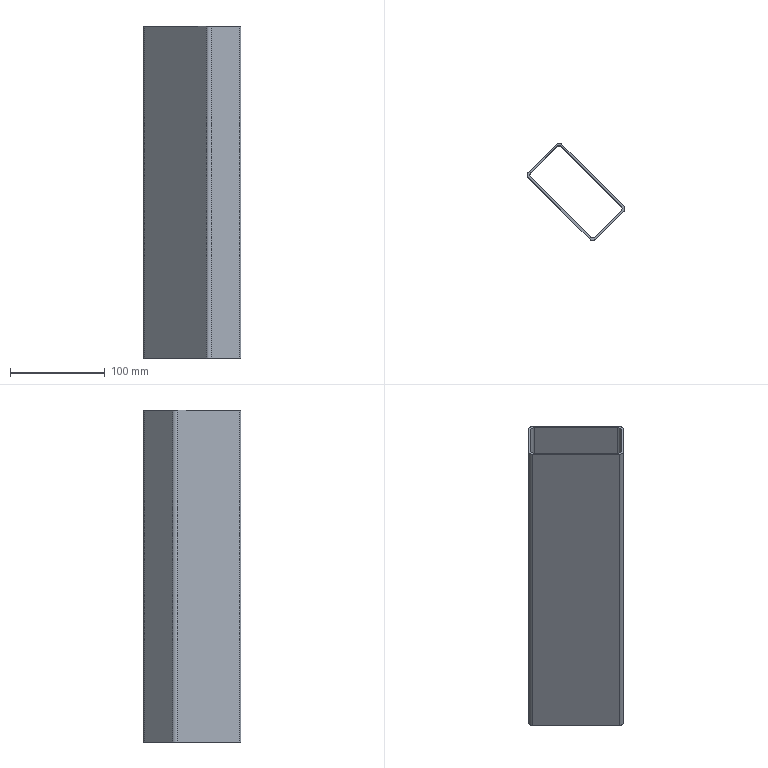Component | NX | SLIDER_FRAME_CONN_BEAM_3 | 1 solid | 18 faces | volume 204400 mm3 | plane 10 | cylinder 8 | commonest cylinder face diameters 8 x8